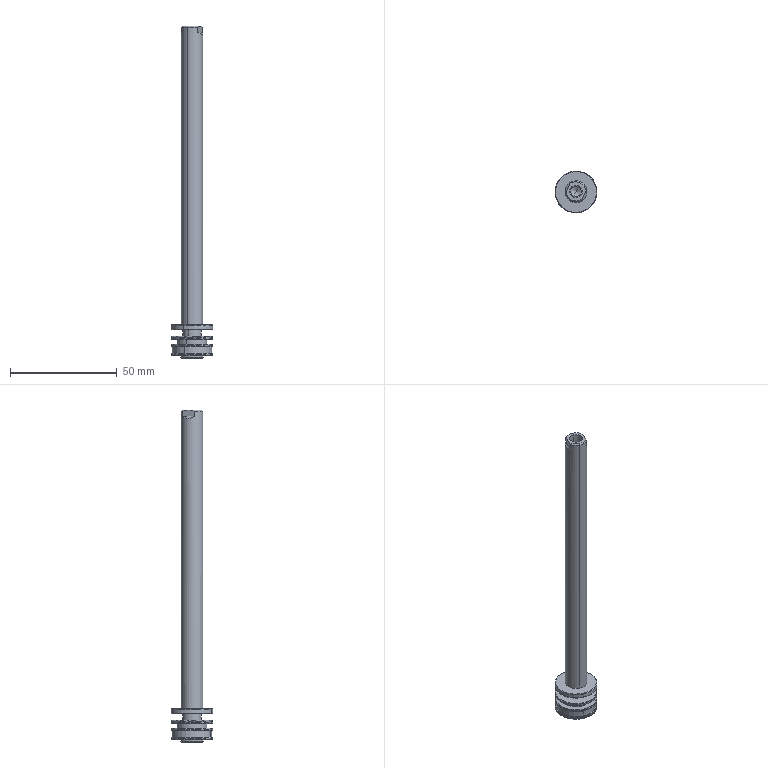Component | SolidWorks | TR-20x75-S-GN-1 (0)-3_TR-20x75-SGuideRod-2 | 1 solid | 60 faces | volume 13841 mm3 | cylinder 22 | cone 19 | plane 15 | spline 4 | commonest cylinder face diameters 19.6 x8 4.917 x2 6 x2 10 x2 8.8 x2 14 x2 18.4 x2 10.6 x2